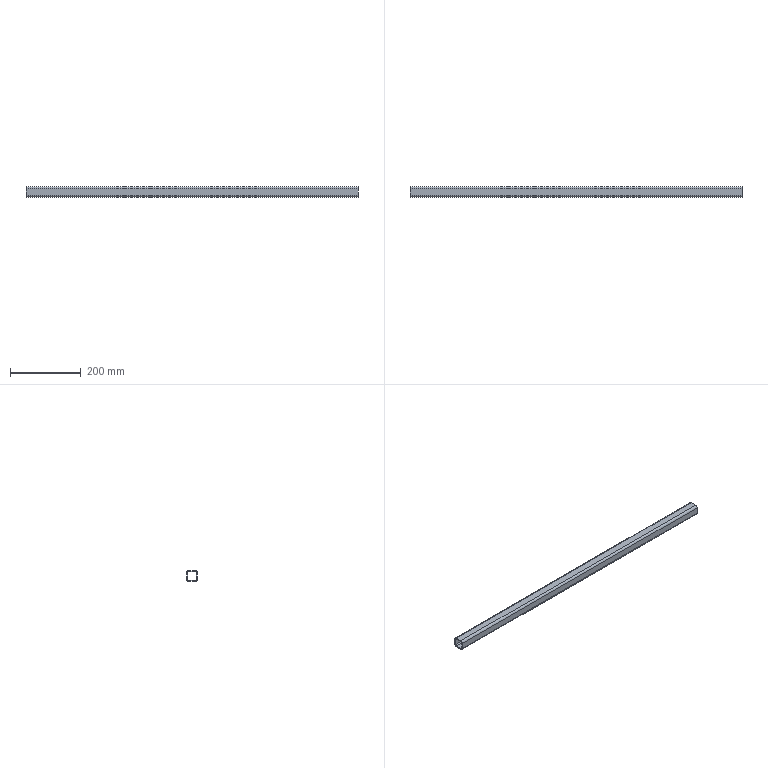Component | SolidWorks | 30X30X3-940-1 | 1 solid | 18 faces | box 940 x 30 x 30 mm | volume 282774 mm3 | plane 10 | cylinder 8 | commonest cylinder face diameters 12 x4 6 x4
build123d program:
from build123d import *

# Parameters (mm, degrees)
GB_6728_1986_SQUARE_HOLLOW_SECTION_030_X_DEPTH = 940


with BuildPart() as part:
    # Sketch1 → Gb_6728-1986 Square Hollow Section 030 X (new body)
    with BuildSketch(Plane(origin=(0, 0, 0), x_dir=(-1, 0, 0), z_dir=(0, 1, 0))):
        with BuildLine():
            Line((-9, -15), (9, -15))
            ThreePointArc((9, -15), (13.243, -13.243), (15, -9))
            Line((15, -9), (15, 9))
            ThreePointArc((15, 9), (13.243, 13.243), (9, 15))
            Line((9, 15), (-9, 15))
            ThreePointArc((-9, 15), (-13.243, 13.243), (-15, 9))
            Line((-15, 9), (-15, -9))
            ThreePointArc((-15, -9), (-13.243, -13.243), (-9, -15))
        make_face()
        with BuildLine():
            Line((-9, -12), (9, -12))
            ThreePointArc((9, -12), (11.121, -11.121), (12, -9))
            Line((12, -9), (12, 9))
            ThreePointArc((12, 9), (11.121, 11.121), (9, 12))
            Line((9, 12), (-9, 12))
            ThreePointArc((-9, 12), (-11.121, 11.121), (-12, 9))
            Line((-12, 9), (-12, -9))
            ThreePointArc((-12, -9), (-11.121, -11.121), (-9, -12))
        make_face(mode=Mode.SUBTRACT)
    extrude(amount=GB_6728_1986_SQUARE_HOLLOW_SECTION_030_X_DEPTH)


solid = part.part

# Placed as in the assembly
solid = solid.moved(Location((3139.926, -31179.846, 3899), (0, 0, 90)))
STEP:
#1=CARTESIAN_POINT('',(86.611,-1227.199,152.913));
#2=VERTEX_POINT('',#1);
#3=CARTESIAN_POINT('',(86.611,-1226.962,153.15));
#4=VERTEX_POINT('',#3);
#5=CARTESIAN_POINT('',(86.611,-1227.199,153.15));
#6=DIRECTION('',(1.,-0.,-0.));
#7=DIRECTION('',(0.,1.,0.));
#8=AXIS2_PLACEMENT_3D('',#5,#6,#7);
#9=CIRCLE('',#8,0.2362);
#10=EDGE_CURVE('',#2,#4,#9,.T.);
#11=ORIENTED_EDGE('',*,*,#10,.T.);
#12=CARTESIAN_POINT('',(123.619,-1226.962,153.15));
#13=VERTEX_POINT('',#12);
#14=CARTESIAN_POINT('',(123.619,-1226.962,153.15));
#15=DIRECTION('',(-1.,0.,0.));
#16=VECTOR('',#15,39.37);
#17=LINE('',#14,#16);
#18=EDGE_CURVE('',#13,#4,#17,.T.);
#19=ORIENTED_EDGE('',*,*,#18,.F.);
#20=CARTESIAN_POINT('',(123.619,-1227.199,152.913));
#21=VERTEX_POINT('',#20);
#22=CARTESIAN_POINT('',(123.619,-1227.199,153.15));
#23=DIRECTION('',(1.,-0.,-0.));
#24=DIRECTION('',(0.,1.,0.));
#25=AXIS2_PLACEMENT_3D('',#22,#23,#24);
#26=CIRCLE('',#25,0.2362);
#27=EDGE_CURVE('',#21,#13,#26,.T.);
#28=ORIENTED_EDGE('',*,*,#27,.F.);
#29=CARTESIAN_POINT('',(123.619,-1227.199,152.913));
#30=DIRECTION('',(-1.,0.,0.));
#31=VECTOR('',#30,39.37);
#32=LINE('',#29,#31);
#33=EDGE_CURVE('',#21,#2,#32,.T.);
#34=ORIENTED_EDGE('',*,*,#33,.T.);
#35=EDGE_LOOP('',(#11,#19,#28,#34));
#36=FACE_OUTER_BOUND('',#35,.T.);
#37=CARTESIAN_POINT('',(123.619,-1227.199,153.15));
#38=DIRECTION('',(-1.,0.,0.));
#39=DIRECTION('',(0.,-1.,0.));
#40=AXIS2_PLACEMENT_3D('',#37,#38,#39);
#41=CYLINDRICAL_SURFACE('',#40,0.2362);
#42=ADVANCED_FACE('',(#36),#41,.T.);
#43=CARTESIAN_POINT('',(86.611,-1226.962,153.858));
#44=VERTEX_POINT('',#43);
#45=CARTESIAN_POINT('',(86.611,-1226.962,153.15));
#46=DIRECTION('',(0.,-0.,1.));
#47=VECTOR('',#46,39.37);
#48=LINE('',#45,#47);
#49=EDGE_CURVE('',#4,#44,#48,.T.);
#50=ORIENTED_EDGE('',*,*,#49,.T.);
#51=CARTESIAN_POINT('',(123.619,-1226.962,153.858));
#52=VERTEX_POINT('',#51);
#53=CARTESIAN_POINT('',(123.619,-1226.962,153.858));
#54=DIRECTION('',(-1.,0.,0.));
#55=VECTOR('',#54,39.37);
#56=LINE('',#53,#55);
#57=EDGE_CURVE('',#52,#44,#56,.T.);
#58=ORIENTED_EDGE('',*,*,#57,.F.);
#59=CARTESIAN_POINT('',(123.619,-1226.962,153.15));
#60=DIRECTION('',(0.,-0.,1.));
#61=VECTOR('',#60,39.37);
#62=LINE('',#59,#61);
#63=EDGE_CURVE('',#13,#52,#62,.T.);
#64=ORIENTED_EDGE('',*,*,#63,.F.);
#65=ORIENTED_EDGE('',*,*,#18,.T.);
#66=EDGE_LOOP('',(#50,#58,#64,#65));
#67=FACE_OUTER_BOUND('',#66,.T.);
#68=CARTESIAN_POINT('',(123.619,-1226.962,153.15));
#69=DIRECTION('',(-0.,-1.,-0.));
#70=DIRECTION('',(-0.,0.,-1.));
#71=AXIS2_PLACEMENT_3D('',#68,#69,#70);
#72=PLANE('',#71);
#73=ADVANCED_FACE('',(#67),#72,.F.);
#74=CARTESIAN_POINT('',(86.611,-1227.199,154.094));
#75=VERTEX_POINT('',#74);
#76=CARTESIAN_POINT('',(86.611,-1227.199,153.858));
#77=DIRECTION('',(1.,-0.,-0.));
#78=DIRECTION('',(0.,1.,0.));
#79=AXIS2_PLACEMENT_3D('',#76,#77,#78);
#80=CIRCLE('',#79,0.2362);
#81=EDGE_CURVE('',#44,#75,#80,.T.);
#82=ORIENTED_EDGE('',*,*,#81,.T.);
#83=CARTESIAN_POINT('',(123.619,-1227.199,154.094));
#84=VERTEX_POINT('',#83);
#85=CARTESIAN_POINT('',(123.619,-1227.199,154.094));
#86=DIRECTION('',(-1.,0.,0.));
#87=VECTOR('',#86,39.37);
#88=LINE('',#85,#87);
#89=EDGE_CURVE('',#84,#75,#88,.T.);
#90=ORIENTED_EDGE('',*,*,#89,.F.);
#91=CARTESIAN_POINT('',(123.619,-1227.199,153.858));
#92=DIRECTION('',(1.,-0.,-0.));
#93=DIRECTION('',(0.,1.,0.));
#94=AXIS2_PLACEMENT_3D('',#91,#92,#93);
#95=CIRCLE('',#94,0.2362);
#96=EDGE_CURVE('',#52,#84,#95,.T.);
#97=ORIENTED_EDGE('',*,*,#96,.F.);
#98=ORIENTED_EDGE('',*,*,#57,.T.);
#99=EDGE_LOOP('',(#82,#90,#97,#98));
#100=FACE_OUTER_BOUND('',#99,.T.);
#101=CARTESIAN_POINT('',(123.619,-1227.199,153.858));
#102=DIRECTION('',(-1.,0.,0.));
#103=DIRECTION('',(0.,-1.,0.));
#104=AXIS2_PLACEMENT_3D('',#101,#102,#103);
#105=CYLINDRICAL_SURFACE('',#104,0.2362);
#106=ADVANCED_FACE('',(#100),#105,.T.);
#107=CARTESIAN_POINT('',(86.611,-1227.907,154.094));
#108=VERTEX_POINT('',#107);
#109=CARTESIAN_POINT('',(86.611,-1227.907,154.094));
#110=DIRECTION('',(-0.,-1.,-0.));
#111=VECTOR('',#110,39.37);
#112=LINE('',#109,#111);
#113=EDGE_CURVE('',#75,#108,#112,.T.);
#114=ORIENTED_EDGE('',*,*,#113,.T.);
#115=CARTESIAN_POINT('',(123.619,-1227.907,154.094));
#116=VERTEX_POINT('',#115);
#117=CARTESIAN_POINT('',(123.619,-1227.907,154.094));
#118=DIRECTION('',(-1.,0.,0.));
#119=VECTOR('',#118,39.37);
#120=LINE('',#117,#119);
#121=EDGE_CURVE('',#116,#108,#120,.T.);
#122=ORIENTED_EDGE('',*,*,#121,.F.);
#123=CARTESIAN_POINT('',(123.619,-1227.907,154.094));
#124=DIRECTION('',(-0.,-1.,-0.));
#125=VECTOR('',#124,39.37);
#126=LINE('',#123,#125);
#127=EDGE_CURVE('',#84,#116,#126,.T.);
#128=ORIENTED_EDGE('',*,*,#127,.F.);
#129=ORIENTED_EDGE('',*,*,#89,.T.);
#130=EDGE_LOOP('',(#114,#122,#128,#129));
#131=FACE_OUTER_BOUND('',#130,.T.);
#132=CARTESIAN_POINT('',(123.619,-1227.907,154.094));
#133=DIRECTION('',(-0.,0.,-1.));
#134=DIRECTION('',(0.,1.,0.));
#135=AXIS2_PLACEMENT_3D('',#132,#133,#134);
#136=PLANE('',#135);
#137=ADVANCED_FACE('',(#131),#136,.F.);
#138=CARTESIAN_POINT('',(86.611,-1228.144,153.858));
#139=VERTEX_POINT('',#138);
#140=CARTESIAN_POINT('',(86.611,-1227.907,153.858));
#141=DIRECTION('',(1.,-0.,-0.));
#142=DIRECTION('',(0.,1.,0.));
#143=AXIS2_PLACEMENT_3D('',#140,#141,#142);
#144=CIRCLE('',#143,0.2362);
#145=EDGE_CURVE('',#108,#139,#144,.T.);
#146=ORIENTED_EDGE('',*,*,#145,.T.);
#147=CARTESIAN_POINT('',(123.619,-1228.144,153.858));
#148=VERTEX_POINT('',#147);
#149=CARTESIAN_POINT('',(123.619,-1228.144,153.858));
#150=DIRECTION('',(-1.,0.,0.));
#151=VECTOR('',#150,39.37);
#152=LINE('',#149,#151);
#153=EDGE_CURVE('',#148,#139,#152,.T.);
#154=ORIENTED_EDGE('',*,*,#153,.F.);
#155=CARTESIAN_POINT('',(123.619,-1227.907,153.858));
#156=DIRECTION('',(1.,-0.,-0.));
#157=DIRECTION('',(0.,1.,0.));
#158=AXIS2_PLACEMENT_3D('',#155,#156,#157);
#159=CIRCLE('',#158,0.2362);
#160=EDGE_CURVE('',#116,#148,#159,.T.);
#161=ORIENTED_EDGE('',*,*,#160,.F.);
#162=ORIENTED_EDGE('',*,*,#121,.T.);
#163=EDGE_LOOP('',(#146,#154,#161,#162));
#164=FACE_OUTER_BOUND('',#163,.T.);
#165=CARTESIAN_POINT('',(123.619,-1227.907,153.858));
#166=DIRECTION('',(-1.,0.,0.));
#167=DIRECTION('',(0.,-1.,0.));
#168=AXIS2_PLACEMENT_3D('',#165,#166,#167);
#169=CYLINDRICAL_SURFACE('',#168,0.2362);
#170=ADVANCED_FACE('',(#164),#169,.T.);
#171=CARTESIAN_POINT('',(86.611,-1228.144,153.15));
#172=VERTEX_POINT('',#171);
#173=CARTESIAN_POINT('',(86.611,-1228.144,153.858));
#174=DIRECTION('',(-0.,0.,-1.));
#175=VECTOR('',#174,39.37);
#176=LINE('',#173,#175);
#177=EDGE_CURVE('',#139,#172,#176,.T.);
#178=ORIENTED_EDGE('',*,*,#177,.T.);
#179=CARTESIAN_POINT('',(123.619,-1228.144,153.15));
#180=VERTEX_POINT('',#179);
#181=CARTESIAN_POINT('',(123.619,-1228.144,153.15));
#182=DIRECTION('',(-1.,0.,0.));
#183=VECTOR('',#182,39.37);
#184=LINE('',#181,#183);
#185=EDGE_CURVE('',#180,#172,#184,.T.);
#186=ORIENTED_EDGE('',*,*,#185,.F.);
#187=CARTESIAN_POINT('',(123.619,-1228.144,153.858));
#188=DIRECTION('',(-0.,0.,-1.));
#189=VECTOR('',#188,39.37);
#190=LINE('',#187,#189);
#191=EDGE_CURVE('',#148,#180,#190,.T.);
#192=ORIENTED_EDGE('',*,*,#191,.F.);
#193=ORIENTED_EDGE('',*,*,#153,.T.);
#194=EDGE_LOOP('',(#178,#186,#192,#193));
#195=FACE_OUTER_BOUND('',#194,.T.);
#196=CARTESIAN_POINT('',(123.619,-1228.144,153.858));
#197=DIRECTION('',(0.,1.,0.));
#198=DIRECTION('',(0.,-0.,1.));
#199=AXIS2_PLACEMENT_3D('',#196,#197,#198);
#200=PLANE('',#199);
#201=ADVANCED_FACE('',(#195),#200,.F.);
#202=CARTESIAN_POINT('',(86.611,-1227.907,152.913));
#203=VERTEX_POINT('',#202);
#204=CARTESIAN_POINT('',(86.611,-1227.907,153.15));
#205=DIRECTION('',(1.,-0.,-0.));
#206=DIRECTION('',(0.,1.,0.));
#207=AXIS2_PLACEMENT_3D('',#204,#205,#206);
#208=CIRCLE('',#207,0.2362);
#209=EDGE_CURVE('',#172,#203,#208,.T.);
#210=ORIENTED_EDGE('',*,*,#209,.T.);
#211=CARTESIAN_POINT('',(123.619,-1227.907,152.913));
#212=VERTEX_POINT('',#211);
#213=CARTESIAN_POINT('',(123.619,-1227.907,152.913));
#214=DIRECTION('',(-1.,0.,0.));
#215=VECTOR('',#214,39.37);
#216=LINE('',#213,#215);
#217=EDGE_CURVE('',#212,#203,#216,.T.);
#218=ORIENTED_EDGE('',*,*,#217,.F.);
#219=CARTESIAN_POINT('',(123.619,-1227.907,153.15));
#220=DIRECTION('',(1.,-0.,-0.));
#221=DIRECTION('',(0.,1.,0.));
#222=AXIS2_PLACEMENT_3D('',#219,#220,#221);
#223=CIRCLE('',#222,0.2362);
#224=EDGE_CURVE('',#180,#212,#223,.T.);
#225=ORIENTED_EDGE('',*,*,#224,.F.);
#226=ORIENTED_EDGE('',*,*,#185,.T.);
#227=EDGE_LOOP('',(#210,#218,#225,#226));
#228=FACE_OUTER_BOUND('',#227,.T.);
#229=CARTESIAN_POINT('',(123.619,-1227.907,153.15));
#230=DIRECTION('',(-1.,0.,0.));
#231=DIRECTION('',(0.,-1.,0.));
#232=AXIS2_PLACEMENT_3D('',#229,#230,#231);
#233=CYLINDRICAL_SURFACE('',#232,0.2362);
#234=ADVANCED_FACE('',(#228),#233,.T.);
#235=CARTESIAN_POINT('',(86.611,-1227.081,153.858));
#236=VERTEX_POINT('',#235);
#237=CARTESIAN_POINT('',(86.611,-1227.199,153.976));
#238=VERTEX_POINT('',#237);
#239=CARTESIAN_POINT('',(86.611,-1227.199,153.858));
#240=DIRECTION('',(1.,-0.,-0.));
#241=DIRECTION('',(0.,1.,0.));
#242=AXIS2_PLACEMENT_3D('',#239,#240,#241);
#243=CIRCLE('',#242,0.1181);
#244=EDGE_CURVE('',#236,#238,#243,.T.);
#245=ORIENTED_EDGE('',*,*,#244,.F.);
#246=CARTESIAN_POINT('',(123.619,-1227.081,153.858));
#247=VERTEX_POINT('',#246);
#248=CARTESIAN_POINT('',(123.619,-1227.081,153.858));
#249=DIRECTION('',(-1.,0.,0.));
#250=VECTOR('',#249,39.37);
#251=LINE('',#248,#250);
#252=EDGE_CURVE('',#247,#236,#251,.T.);
#253=ORIENTED_EDGE('',*,*,#252,.F.);
#254=CARTESIAN_POINT('',(123.619,-1227.199,153.976));
#255=VERTEX_POINT('',#254);
#256=CARTESIAN_POINT('',(123.619,-1227.199,153.858));
#257=DIRECTION('',(1.,-0.,-0.));
#258=DIRECTION('',(0.,1.,0.));
#259=AXIS2_PLACEMENT_3D('',#256,#257,#258);
#260=CIRCLE('',#259,0.1181);
#261=EDGE_CURVE('',#247,#255,#260,.T.);
#262=ORIENTED_EDGE('',*,*,#261,.T.);
#263=CARTESIAN_POINT('',(123.619,-1227.199,153.976));
#264=DIRECTION('',(-1.,0.,0.));
#265=VECTOR('',#264,39.37);
#266=LINE('',#263,#265);
#267=EDGE_CURVE('',#255,#238,#266,.T.);
#268=ORIENTED_EDGE('',*,*,#267,.T.);
#269=EDGE_LOOP('',(#245,#253,#262,#268));
#270=FACE_OUTER_BOUND('',#269,.T.);
#271=CARTESIAN_POINT('',(123.619,-1227.199,153.858));
#272=DIRECTION('',(-1.,0.,0.));
#273=DIRECTION('',(0.,-1.,0.));
#274=AXIS2_PLACEMENT_3D('',#271,#272,#273);
#275=CYLINDRICAL_SURFACE('',#274,0.1181);
#276=ADVANCED_FACE('',(#270),#275,.F.);
#277=CARTESIAN_POINT('',(86.611,-1227.081,153.15));
#278=VERTEX_POINT('',#277);
#279=CARTESIAN_POINT('',(86.611,-1227.081,153.15));
#280=DIRECTION('',(0.,-0.,1.));
#281=VECTOR('',#280,39.37);
#282=LINE('',#279,#281);
#283=EDGE_CURVE('',#278,#236,#282,.T.);
#284=ORIENTED_EDGE('',*,*,#283,.F.);
#285=CARTESIAN_POINT('',(123.619,-1227.081,153.15));
#286=VERTEX_POINT('',#285);
#287=CARTESIAN_POINT('',(123.619,-1227.081,153.15));
#288=DIRECTION('',(-1.,0.,0.));
#289=VECTOR('',#288,39.37);
#290=LINE('',#287,#289);
#291=EDGE_CURVE('',#286,#278,#290,.T.);
#292=ORIENTED_EDGE('',*,*,#291,.F.);
#293=CARTESIAN_POINT('',(123.619,-1227.081,153.15));
#294=DIRECTION('',(0.,-0.,1.));
#295=VECTOR('',#294,39.37);
#296=LINE('',#293,#295);
#297=EDGE_CURVE('',#286,#247,#296,.T.);
#298=ORIENTED_EDGE('',*,*,#297,.T.);
#299=ORIENTED_EDGE('',*,*,#252,.T.);
#300=EDGE_LOOP('',(#284,#292,#298,#299));
#301=FACE_OUTER_BOUND('',#300,.T.);
#302=CARTESIAN_POINT('',(123.619,-1227.081,153.15));
#303=DIRECTION('',(-0.,-1.,-0.));
#304=DIRECTION('',(-0.,0.,-1.));
#305=AXIS2_PLACEMENT_3D('',#302,#303,#304);
#306=PLANE('',#305);
#307=ADVANCED_FACE('',(#301),#306,.T.);
#308=CARTESIAN_POINT('',(86.611,-1227.199,153.031));
#309=VERTEX_POINT('',#308);
#310=CARTESIAN_POINT('',(86.611,-1227.199,153.15));
#311=DIRECTION('',(1.,-0.,-0.));
#312=DIRECTION('',(0.,1.,0.));
#313=AXIS2_PLACEMENT_3D('',#310,#311,#312);
#314=CIRCLE('',#313,0.1181);
#315=EDGE_CURVE('',#309,#278,#314,.T.);
#316=ORIENTED_EDGE('',*,*,#315,.F.);
#317=CARTESIAN_POINT('',(123.619,-1227.199,153.031));
#318=VERTEX_POINT('',#317);
#319=CARTESIAN_POINT('',(123.619,-1227.199,153.031));
#320=DIRECTION('',(-1.,0.,0.));
#321=VECTOR('',#320,39.37);
#322=LINE('',#319,#321);
#323=EDGE_CURVE('',#318,#309,#322,.T.);
#324=ORIENTED_EDGE('',*,*,#323,.F.);
#325=CARTESIAN_POINT('',(123.619,-1227.199,153.15));
#326=DIRECTION('',(1.,-0.,-0.));
#327=DIRECTION('',(0.,1.,0.));
#328=AXIS2_PLACEMENT_3D('',#325,#326,#327);
#329=CIRCLE('',#328,0.1181);
#330=EDGE_CURVE('',#318,#286,#329,.T.);
#331=ORIENTED_EDGE('',*,*,#330,.T.);
#332=ORIENTED_EDGE('',*,*,#291,.T.);
#333=EDGE_LOOP('',(#316,#324,#331,#332));
#334=FACE_OUTER_BOUND('',#333,.T.);
#335=CARTESIAN_POINT('',(123.619,-1227.199,153.15));
#336=DIRECTION('',(-1.,0.,0.));
#337=DIRECTION('',(0.,-1.,0.));
#338=AXIS2_PLACEMENT_3D('',#335,#336,#337);
#339=CYLINDRICAL_SURFACE('',#338,0.1181);
#340=ADVANCED_FACE('',(#334),#339,.F.);
#341=CARTESIAN_POINT('',(86.611,-1227.907,153.031));
#342=VERTEX_POINT('',#341);
#343=CARTESIAN_POINT('',(86.611,-1227.199,153.031));
#344=DIRECTION('',(0.,1.,0.));
#345=VECTOR('',#344,39.37);
#346=LINE('',#343,#345);
#347=EDGE_CURVE('',#342,#309,#346,.T.);
#348=ORIENTED_EDGE('',*,*,#347,.F.);
#349=CARTESIAN_POINT('',(123.619,-1227.907,153.031));
#350=VERTEX_POINT('',#349);
#351=CARTESIAN_POINT('',(123.619,-1227.907,153.031));
#352=DIRECTION('',(-1.,0.,0.));
#353=VECTOR('',#352,39.37);
#354=LINE('',#351,#353);
#355=EDGE_CURVE('',#350,#342,#354,.T.);
#356=ORIENTED_EDGE('',*,*,#355,.F.);
#357=CARTESIAN_POINT('',(123.619,-1227.199,153.031));
#358=DIRECTION('',(0.,1.,0.));
#359=VECTOR('',#358,39.37);
#360=LINE('',#357,#359);
#361=EDGE_CURVE('',#350,#318,#360,.T.);
#362=ORIENTED_EDGE('',*,*,#361,.T.);
#363=ORIENTED_EDGE('',*,*,#323,.T.);
#364=EDGE_LOOP('',(#348,#356,#362,#363));
#365=FACE_OUTER_BOUND('',#364,.T.);
#366=CARTESIAN_POINT('',(123.619,-1227.199,153.031));
#367=DIRECTION('',(0.,-0.,1.));
#368=DIRECTION('',(-0.,-1.,-0.));
#369=AXIS2_PLACEMENT_3D('',#366,#367,#368);
#370=PLANE('',#369);
#371=ADVANCED_FACE('',(#365),#370,.T.);
#372=CARTESIAN_POINT('',(86.611,-1228.025,153.15));
#373=VERTEX_POINT('',#372);
#374=CARTESIAN_POINT('',(86.611,-1227.907,153.15));
#375=DIRECTION('',(1.,-0.,-0.));
#376=DIRECTION('',(0.,1.,0.));
#377=AXIS2_PLACEMENT_3D('',#374,#375,#376);
#378=CIRCLE('',#377,0.1181);
#379=EDGE_CURVE('',#373,#342,#378,.T.);
#380=ORIENTED_EDGE('',*,*,#379,.F.);
#381=CARTESIAN_POINT('',(123.619,-1228.025,153.15));
#382=VERTEX_POINT('',#381);
#383=CARTESIAN_POINT('',(123.619,-1228.025,153.15));
#384=DIRECTION('',(-1.,0.,0.));
#385=VECTOR('',#384,39.37);
#386=LINE('',#383,#385);
#387=EDGE_CURVE('',#382,#373,#386,.T.);
#388=ORIENTED_EDGE('',*,*,#387,.F.);
#389=CARTESIAN_POINT('',(123.619,-1227.907,153.15));
#390=DIRECTION('',(1.,-0.,-0.));
#391=DIRECTION('',(0.,1.,0.));
#392=AXIS2_PLACEMENT_3D('',#389,#390,#391);
#393=CIRCLE('',#392,0.1181);
#394=EDGE_CURVE('',#382,#350,#393,.T.);
#395=ORIENTED_EDGE('',*,*,#394,.T.);
#396=ORIENTED_EDGE('',*,*,#355,.T.);
#397=EDGE_LOOP('',(#380,#388,#395,#396));
#398=FACE_OUTER_BOUND('',#397,.T.);
#399=CARTESIAN_POINT('',(123.619,-1227.907,153.15));
#400=DIRECTION('',(-1.,0.,0.));
#401=DIRECTION('',(0.,-1.,0.));
#402=AXIS2_PLACEMENT_3D('',#399,#400,#401);
#403=CYLINDRICAL_SURFACE('',#402,0.1181);
#404=ADVANCED_FACE('',(#398),#403,.F.);
#405=CARTESIAN_POINT('',(86.611,-1228.025,153.858));
#406=VERTEX_POINT('',#405);
#407=CARTESIAN_POINT('',(86.611,-1228.025,153.858));
#408=DIRECTION('',(-0.,0.,-1.));
#409=VECTOR('',#408,39.37);
#410=LINE('',#407,#409);
#411=EDGE_CURVE('',#406,#373,#410,.T.);
#412=ORIENTED_EDGE('',*,*,#411,.F.);
#413=CARTESIAN_POINT('',(123.619,-1228.025,153.858));
#414=VERTEX_POINT('',#413);
#415=CARTESIAN_POINT('',(123.619,-1228.025,153.858));
#416=DIRECTION('',(-1.,0.,0.));
#417=VECTOR('',#416,39.37);
#418=LINE('',#415,#417);
#419=EDGE_CURVE('',#414,#406,#418,.T.);
#420=ORIENTED_EDGE('',*,*,#419,.F.);
#421=CARTESIAN_POINT('',(123.619,-1228.025,153.858));
#422=DIRECTION('',(-0.,0.,-1.));
#423=VECTOR('',#422,39.37);
#424=LINE('',#421,#423);
#425=EDGE_CURVE('',#414,#382,#424,.T.);
#426=ORIENTED_EDGE('',*,*,#425,.T.);
#427=ORIENTED_EDGE('',*,*,#387,.T.);
#428=EDGE_LOOP('',(#412,#420,#426,#427));
#429=FACE_OUTER_BOUND('',#428,.T.);
#430=CARTESIAN_POINT('',(123.619,-1228.025,153.858));
#431=DIRECTION('',(0.,1.,0.));
#432=DIRECTION('',(0.,-0.,1.));
#433=AXIS2_PLACEMENT_3D('',#430,#431,#432);
#434=PLANE('',#433);
#435=ADVANCED_FACE('',(#429),#434,.T.);
#436=CARTESIAN_POINT('',(86.611,-1227.907,153.976));
#437=VERTEX_POINT('',#436);
#438=CARTESIAN_POINT('',(86.611,-1227.907,153.858));
#439=DIRECTION('',(1.,-0.,-0.));
#440=DIRECTION('',(0.,1.,0.));
#441=AXIS2_PLACEMENT_3D('',#438,#439,#440);
#442=CIRCLE('',#441,0.1181);
#443=EDGE_CURVE('',#437,#406,#442,.T.);
#444=ORIENTED_EDGE('',*,*,#443,.F.);
#445=CARTESIAN_POINT('',(123.619,-1227.907,153.976));
#446=VERTEX_POINT('',#445);
#447=CARTESIAN_POINT('',(123.619,-1227.907,153.976));
#448=DIRECTION('',(-1.,0.,0.));
#449=VECTOR('',#448,39.37);
#450=LINE('',#447,#449);
#451=EDGE_CURVE('',#446,#437,#450,.T.);
#452=ORIENTED_EDGE('',*,*,#451,.F.);
#453=CARTESIAN_POINT('',(123.619,-1227.907,153.858));
#454=DIRECTION('',(1.,-0.,-0.));
#455=DIRECTION('',(0.,1.,0.));
#456=AXIS2_PLACEMENT_3D('',#453,#454,#455);
#457=CIRCLE('',#456,0.1181);
#458=EDGE_CURVE('',#446,#414,#457,.T.);
#459=ORIENTED_EDGE('',*,*,#458,.T.);
#460=ORIENTED_EDGE('',*,*,#419,.T.);
#461=EDGE_LOOP('',(#444,#452,#459,#460));
#462=FACE_OUTER_BOUND('',#461,.T.);
#463=CARTESIAN_POINT('',(123.619,-1227.907,153.858));
#464=DIRECTION('',(-1.,0.,0.));
#465=DIRECTION('',(0.,-1.,0.));
#466=AXIS2_PLACEMENT_3D('',#463,#464,#465);
#467=CYLINDRICAL_SURFACE('',#466,0.1181);
#468=ADVANCED_FACE('',(#462),#467,.F.);
#469=CARTESIAN_POINT('',(86.611,-1227.907,153.976));
#470=DIRECTION('',(-0.,-1.,-0.));
#471=VECTOR('',#470,39.37);
#472=LINE('',#469,#471);
#473=EDGE_CURVE('',#238,#437,#472,.T.);
#474=ORIENTED_EDGE('',*,*,#473,.F.);
#475=ORIENTED_EDGE('',*,*,#267,.F.);
#476=CARTESIAN_POINT('',(123.619,-1227.907,153.976));
#477=DIRECTION('',(-0.,-1.,-0.));
#478=VECTOR('',#477,39.37);
#479=LINE('',#476,#478);
#480=EDGE_CURVE('',#255,#446,#479,.T.);
#481=ORIENTED_EDGE('',*,*,#480,.T.);
#482=ORIENTED_EDGE('',*,*,#451,.T.);
#483=EDGE_LOOP('',(#474,#475,#481,#482));
#484=FACE_OUTER_BOUND('',#483,.T.);
#485=CARTESIAN_POINT('',(123.619,-1227.907,153.976));
#486=DIRECTION('',(-0.,0.,-1.));
#487=DIRECTION('',(0.,1.,0.));
#488=AXIS2_PLACEMENT_3D('',#485,#486,#487);
#489=PLANE('',#488);
#490=ADVANCED_FACE('',(#484),#489,.T.);
#491=CARTESIAN_POINT('',(86.611,-1227.199,152.913));
#492=DIRECTION('',(0.,1.,0.));
#493=VECTOR('',#492,39.37);
#494=LINE('',#491,#493);
#495=EDGE_CURVE('',#203,#2,#494,.T.);
#496=ORIENTED_EDGE('',*,*,#495,.T.);
#497=ORIENTED_EDGE('',*,*,#33,.F.);
#498=CARTESIAN_POINT('',(123.619,-1227.199,152.913));
#499=DIRECTION('',(0.,1.,0.));
#500=VECTOR('',#499,39.37);
#501=LINE('',#498,#500);
#502=EDGE_CURVE('',#212,#21,#501,.T.);
#503=ORIENTED_EDGE('',*,*,#502,.F.);
#504=ORIENTED_EDGE('',*,*,#217,.T.);
#505=EDGE_LOOP('',(#496,#497,#503,#504));
#506=FACE_OUTER_BOUND('',#505,.T.);
#507=CARTESIAN_POINT('',(123.619,-1227.199,152.913));
#508=DIRECTION('',(0.,-0.,1.));
#509=DIRECTION('',(-0.,-1.,-0.));
#510=AXIS2_PLACEMENT_3D('',#507,#508,#509);
#511=PLANE('',#510);
#512=ADVANCED_FACE('',(#506),#511,.F.);
#513=ORIENTED_EDGE('',*,*,#261,.F.);
#514=ORIENTED_EDGE('',*,*,#297,.F.);
#515=ORIENTED_EDGE('',*,*,#330,.F.);
#516=ORIENTED_EDGE('',*,*,#361,.F.);
#517=ORIENTED_EDGE('',*,*,#394,.F.);
#518=ORIENTED_EDGE('',*,*,#425,.F.);
#519=ORIENTED_EDGE('',*,*,#458,.F.);
#520=ORIENTED_EDGE('',*,*,#480,.F.);
#521=EDGE_LOOP('',(#513,#514,#515,#516,#517,#518,#519,#520));
#522=FACE_BOUND('',#521,.T.);
#523=ORIENTED_EDGE('',*,*,#27,.T.);
#524=ORIENTED_EDGE('',*,*,#63,.T.);
#525=ORIENTED_EDGE('',*,*,#96,.T.);
#526=ORIENTED_EDGE('',*,*,#127,.T.);
#527=ORIENTED_EDGE('',*,*,#160,.T.);
#528=ORIENTED_EDGE('',*,*,#191,.T.);
#529=ORIENTED_EDGE('',*,*,#224,.T.);
#530=ORIENTED_EDGE('',*,*,#502,.T.);
#531=EDGE_LOOP('',(#523,#524,#525,#526,#527,#528,#529,#530));
#532=FACE_OUTER_BOUND('',#531,.T.);
#533=CARTESIAN_POINT('',(123.619,-1227.199,153.15));
#534=DIRECTION('',(1.,-0.,-0.));
#535=DIRECTION('',(0.,1.,0.));
#536=AXIS2_PLACEMENT_3D('',#533,#534,#535);
#537=PLANE('',#536);
#538=ADVANCED_FACE('',(#522,#532),#537,.T.);
#539=ORIENTED_EDGE('',*,*,#244,.T.);
#540=ORIENTED_EDGE('',*,*,#473,.T.);
#541=ORIENTED_EDGE('',*,*,#443,.T.);
#542=ORIENTED_EDGE('',*,*,#411,.T.);
#543=ORIENTED_EDGE('',*,*,#379,.T.);
#544=ORIENTED_EDGE('',*,*,#347,.T.);
#545=ORIENTED_EDGE('',*,*,#315,.T.);
#546=ORIENTED_EDGE('',*,*,#283,.T.);
#547=EDGE_LOOP('',(#539,#540,#541,#542,#543,#544,#545,#546));
#548=FACE_BOUND('',#547,.T.);
#549=ORIENTED_EDGE('',*,*,#10,.F.);
#550=ORIENTED_EDGE('',*,*,#495,.F.);
#551=ORIENTED_EDGE('',*,*,#209,.F.);
#552=ORIENTED_EDGE('',*,*,#177,.F.);
#553=ORIENTED_EDGE('',*,*,#145,.F.);
#554=ORIENTED_EDGE('',*,*,#113,.F.);
#555=ORIENTED_EDGE('',*,*,#81,.F.);
#556=ORIENTED_EDGE('',*,*,#49,.F.);
#557=EDGE_LOOP('',(#549,#550,#551,#552,#553,#554,#555,#556));
#558=FACE_OUTER_BOUND('',#557,.T.);
#559=CARTESIAN_POINT('',(86.611,-1227.199,153.15));
#560=DIRECTION('',(1.,-0.,-0.));
#561=DIRECTION('',(0.,1.,0.));
#562=AXIS2_PLACEMENT_3D('',#559,#560,#561);
#563=PLANE('',#562);
#564=ADVANCED_FACE('',(#548,#558),#563,.F.);
#565=CLOSED_SHELL('',(#42,#73,#106,#137,#170,#201,#234,#276,#307,#340,#371,#404,#435,#468,#490,#512,#538,#564));
#566=MANIFOLD_SOLID_BREP('',#565);
#567=CARTESIAN_POINT('',(0.,0.,0.));
#568=DIRECTION('',(0.,0.,1.));
#569=DIRECTION('',(1.,0.,0.));
#570=AXIS2_PLACEMENT_3D('',#567,#568,#569);
#571=(LENGTH_UNIT()NAMED_UNIT(*)SI_UNIT($,.METRE.));
#572=LENGTH_MEASURE_WITH_UNIT(LENGTH_MEASURE(0.0254),#571);
#573=DIMENSIONAL_EXPONENTS(1.,0.,0.,0.,0.,0.,0.);
#574=(CONVERSION_BASED_UNIT('',#572)LENGTH_UNIT()NAMED_UNIT(#573));
#575=UNCERTAINTY_MEASURE_WITH_UNIT(LENGTH_MEASURE(0.00001),#574,'','');
#576=(NAMED_UNIT(*)PLANE_ANGLE_UNIT()SI_UNIT($,.RADIAN.));
#577=(NAMED_UNIT(*)SI_UNIT($,.STERADIAN.)SOLID_ANGLE_UNIT());
#578=(GEOMETRIC_REPRESENTATION_CONTEXT(3)GLOBAL_UNCERTAINTY_ASSIGNED_CONTEXT((#575))GLOBAL_UNIT_ASSIGNED_CONTEXT((#574,#576,#577))REPRESENTATION_CONTEXT('',''));
#579=ADVANCED_BREP_SHAPE_REPRESENTATION('',(#566,#570),#578);
#580=COLOUR_RGB('',0.7922,0.8196,0.9333);
#581=FILL_AREA_STYLE_COLOUR('',#580);
#582=FILL_AREA_STYLE('',(#581));
#583=SURFACE_STYLE_FILL_AREA(#582);
#584=SURFACE_SIDE_STYLE('',(#583));
#585=SURFACE_STYLE_USAGE(.BOTH.,#584);
#586=PRESENTATION_STYLE_ASSIGNMENT((#585));
#587=STYLED_ITEM('',(#586),#566);
#588=PRESENTATION_LAYER_ASSIGNMENT('','',(#587));
#589=(LENGTH_UNIT()NAMED_UNIT(*)SI_UNIT($,.METRE.));
#590=LENGTH_MEASURE_WITH_UNIT(LENGTH_MEASURE(0.0254),#589);
#591=DIMENSIONAL_EXPONENTS(1.,0.,0.,0.,0.,0.,0.);
#592=(CONVERSION_BASED_UNIT('',#590)LENGTH_UNIT()NAMED_UNIT(#591));
#593=UNCERTAINTY_MEASURE_WITH_UNIT(LENGTH_MEASURE(0.00001),#592,'','');
#594=(NAMED_UNIT(*)PLANE_ANGLE_UNIT()SI_UNIT($,.RADIAN.));
#595=(NAMED_UNIT(*)SI_UNIT($,.STERADIAN.)SOLID_ANGLE_UNIT());
#596=(GEOMETRIC_REPRESENTATION_CONTEXT(3)GLOBAL_UNCERTAINTY_ASSIGNED_CONTEXT((#593))GLOBAL_UNIT_ASSIGNED_CONTEXT((#592,#594,#595))REPRESENTATION_CONTEXT('',''));
#597=MECHANICAL_DESIGN_GEOMETRIC_PRESENTATION_REPRESENTATION('',(#587),#596);